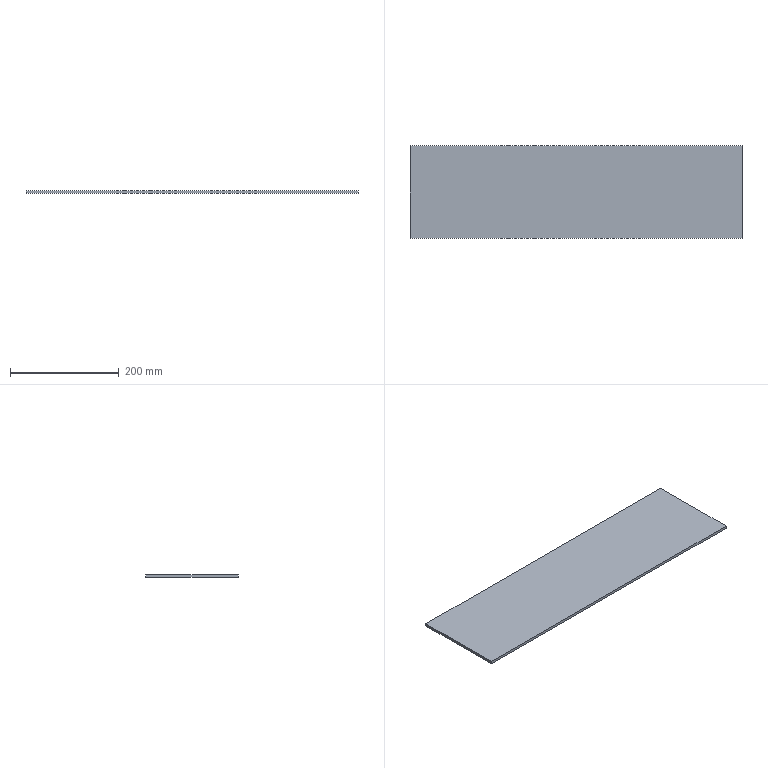Component | SolidWorks | CoverPlate5-1 | 1 solid | 6 faces | box 610 x 170 x 5 mm | volume 518500 mm3 | plane 6
build123d program:
from build123d import *

# Parameters (mm, degrees)
SKETCH1_W      = 610
SKETCH1_H      = 170
EXTRUDE1_DEPTH = 5


with BuildPart() as part:
    # Sketch1 → Extrude1 (new body)
    with BuildSketch(Plane.XY):
        Rectangle(SKETCH1_W, SKETCH1_H)
    extrude(amount=EXTRUDE1_DEPTH)


solid = part.part

# Placed as in the assembly
solid = solid.moved(Location((15, 530, -25), (0, 0, 0)))
STEP:
#1=COLOUR_RGB('',0.7922,0.8196,0.9333);
#2=FILL_AREA_STYLE_COLOUR('',#1);
#3=FILL_AREA_STYLE('',(#2));
#4=SURFACE_STYLE_FILL_AREA(#3);
#5=SURFACE_SIDE_STYLE('',(#4));
#6=SURFACE_STYLE_USAGE(.BOTH.,#5);
#7=PRESENTATION_STYLE_ASSIGNMENT((#6));
#8=CARTESIAN_POINT('',(12.598,17.52,-0.9843));
#9=VERTEX_POINT('',#8);
#10=CARTESIAN_POINT('',(12.598,24.213,-0.9843));
#11=VERTEX_POINT('',#10);
#12=CARTESIAN_POINT('',(12.598,24.213,-0.9843));
#13=DIRECTION('',(0.,1.,0.));
#14=VECTOR('',#13,39.37);
#15=LINE('',#12,#14);
#16=EDGE_CURVE('',#9,#11,#15,.T.);
#17=ORIENTED_EDGE('',*,*,#16,.T.);
#18=CARTESIAN_POINT('',(12.598,24.213,-0.7874));
#19=VERTEX_POINT('',#18);
#20=CARTESIAN_POINT('',(12.598,24.213,-0.7874));
#21=DIRECTION('',(0.,0.,-1.));
#22=VECTOR('',#21,39.37);
#23=LINE('',#20,#22);
#24=EDGE_CURVE('',#19,#11,#23,.T.);
#25=ORIENTED_EDGE('',*,*,#24,.F.);
#26=CARTESIAN_POINT('',(12.598,17.52,-0.7874));
#27=VERTEX_POINT('',#26);
#28=CARTESIAN_POINT('',(12.598,24.213,-0.7874));
#29=DIRECTION('',(0.,1.,0.));
#30=VECTOR('',#29,39.37);
#31=LINE('',#28,#30);
#32=EDGE_CURVE('',#27,#19,#31,.T.);
#33=ORIENTED_EDGE('',*,*,#32,.F.);
#34=CARTESIAN_POINT('',(12.598,17.52,-0.7874));
#35=DIRECTION('',(0.,0.,-1.));
#36=VECTOR('',#35,39.37);
#37=LINE('',#34,#36);
#38=EDGE_CURVE('',#27,#9,#37,.T.);
#39=ORIENTED_EDGE('',*,*,#38,.T.);
#40=EDGE_LOOP('',(#17,#25,#33,#39));
#41=FACE_OUTER_BOUND('',#40,.T.);
#42=CARTESIAN_POINT('',(12.598,24.213,-0.7874));
#43=DIRECTION('',(-1.,0.,0.));
#44=DIRECTION('',(0.,0.,1.));
#45=AXIS2_PLACEMENT_3D('',#42,#43,#44);
#46=PLANE('',#45);
#47=ADVANCED_FACE('',(#41),#46,.F.);
#48=CARTESIAN_POINT('',(-11.417,24.213,-0.9843));
#49=VERTEX_POINT('',#48);
#50=CARTESIAN_POINT('',(-11.417,24.213,-0.9843));
#51=DIRECTION('',(-1.,0.,0.));
#52=VECTOR('',#51,39.37);
#53=LINE('',#50,#52);
#54=EDGE_CURVE('',#11,#49,#53,.T.);
#55=ORIENTED_EDGE('',*,*,#54,.T.);
#56=CARTESIAN_POINT('',(-11.417,24.213,-0.7874));
#57=VERTEX_POINT('',#56);
#58=CARTESIAN_POINT('',(-11.417,24.213,-0.7874));
#59=DIRECTION('',(0.,0.,-1.));
#60=VECTOR('',#59,39.37);
#61=LINE('',#58,#60);
#62=EDGE_CURVE('',#57,#49,#61,.T.);
#63=ORIENTED_EDGE('',*,*,#62,.F.);
#64=CARTESIAN_POINT('',(-11.417,24.213,-0.7874));
#65=DIRECTION('',(-1.,0.,0.));
#66=VECTOR('',#65,39.37);
#67=LINE('',#64,#66);
#68=EDGE_CURVE('',#19,#57,#67,.T.);
#69=ORIENTED_EDGE('',*,*,#68,.F.);
#70=ORIENTED_EDGE('',*,*,#24,.T.);
#71=EDGE_LOOP('',(#55,#63,#69,#70));
#72=FACE_OUTER_BOUND('',#71,.T.);
#73=CARTESIAN_POINT('',(-11.417,24.213,-0.7874));
#74=DIRECTION('',(0.,-1.,0.));
#75=DIRECTION('',(0.,0.,-1.));
#76=AXIS2_PLACEMENT_3D('',#73,#74,#75);
#77=PLANE('',#76);
#78=ADVANCED_FACE('',(#72),#77,.F.);
#79=CARTESIAN_POINT('',(-11.417,17.52,-0.9843));
#80=VERTEX_POINT('',#79);
#81=CARTESIAN_POINT('',(-11.417,24.213,-0.9843));
#82=DIRECTION('',(-0.,-1.,0.));
#83=VECTOR('',#82,39.37);
#84=LINE('',#81,#83);
#85=EDGE_CURVE('',#49,#80,#84,.T.);
#86=ORIENTED_EDGE('',*,*,#85,.T.);
#87=CARTESIAN_POINT('',(-11.417,17.52,-0.7874));
#88=VERTEX_POINT('',#87);
#89=CARTESIAN_POINT('',(-11.417,17.52,-0.7874));
#90=DIRECTION('',(0.,0.,-1.));
#91=VECTOR('',#90,39.37);
#92=LINE('',#89,#91);
#93=EDGE_CURVE('',#88,#80,#92,.T.);
#94=ORIENTED_EDGE('',*,*,#93,.F.);
#95=CARTESIAN_POINT('',(-11.417,24.213,-0.7874));
#96=DIRECTION('',(-0.,-1.,0.));
#97=VECTOR('',#96,39.37);
#98=LINE('',#95,#97);
#99=EDGE_CURVE('',#57,#88,#98,.T.);
#100=ORIENTED_EDGE('',*,*,#99,.F.);
#101=ORIENTED_EDGE('',*,*,#62,.T.);
#102=EDGE_LOOP('',(#86,#94,#100,#101));
#103=FACE_OUTER_BOUND('',#102,.T.);
#104=CARTESIAN_POINT('',(-11.417,24.213,-0.7874));
#105=DIRECTION('',(1.,-0.,0.));
#106=DIRECTION('',(0.,1.,0.));
#107=AXIS2_PLACEMENT_3D('',#104,#105,#106);
#108=PLANE('',#107);
#109=ADVANCED_FACE('',(#103),#108,.F.);
#110=CARTESIAN_POINT('',(-11.417,17.52,-0.9843));
#111=DIRECTION('',(1.,0.,0.));
#112=VECTOR('',#111,39.37);
#113=LINE('',#110,#112);
#114=EDGE_CURVE('',#80,#9,#113,.T.);
#115=ORIENTED_EDGE('',*,*,#114,.T.);
#116=ORIENTED_EDGE('',*,*,#38,.F.);
#117=CARTESIAN_POINT('',(-11.417,17.52,-0.7874));
#118=DIRECTION('',(1.,0.,0.));
#119=VECTOR('',#118,39.37);
#120=LINE('',#117,#119);
#121=EDGE_CURVE('',#88,#27,#120,.T.);
#122=ORIENTED_EDGE('',*,*,#121,.F.);
#123=ORIENTED_EDGE('',*,*,#93,.T.);
#124=EDGE_LOOP('',(#115,#116,#122,#123));
#125=FACE_OUTER_BOUND('',#124,.T.);
#126=CARTESIAN_POINT('',(-11.417,17.52,-0.7874));
#127=DIRECTION('',(0.,1.,0.));
#128=DIRECTION('',(0.,0.,1.));
#129=AXIS2_PLACEMENT_3D('',#126,#127,#128);
#130=PLANE('',#129);
#131=ADVANCED_FACE('',(#125),#130,.F.);
#132=ORIENTED_EDGE('',*,*,#32,.T.);
#133=ORIENTED_EDGE('',*,*,#68,.T.);
#134=ORIENTED_EDGE('',*,*,#99,.T.);
#135=ORIENTED_EDGE('',*,*,#121,.T.);
#136=EDGE_LOOP('',(#132,#133,#134,#135));
#137=FACE_OUTER_BOUND('',#136,.T.);
#138=CARTESIAN_POINT('',(0.5906,20.866,-0.7874));
#139=DIRECTION('',(0.,0.,1.));
#140=DIRECTION('',(1.,0.,0.));
#141=AXIS2_PLACEMENT_3D('',#138,#139,#140);
#142=PLANE('',#141);
#143=ADVANCED_FACE('',(#137),#142,.T.);
#144=ORIENTED_EDGE('',*,*,#16,.F.);
#145=ORIENTED_EDGE('',*,*,#114,.F.);
#146=ORIENTED_EDGE('',*,*,#85,.F.);
#147=ORIENTED_EDGE('',*,*,#54,.F.);
#148=EDGE_LOOP('',(#144,#145,#146,#147));
#149=FACE_OUTER_BOUND('',#148,.T.);
#150=CARTESIAN_POINT('',(0.5906,20.866,-0.9843));
#151=DIRECTION('',(0.,0.,1.));
#152=DIRECTION('',(1.,0.,0.));
#153=AXIS2_PLACEMENT_3D('',#150,#151,#152);
#154=PLANE('',#153);
#155=ADVANCED_FACE('',(#149),#154,.F.);
#156=CLOSED_SHELL('',(#47,#78,#109,#131,#143,#155));
#157=MANIFOLD_SOLID_BREP('',#156);
#158=STYLED_ITEM('',(#7),#157);
#159=(LENGTH_UNIT()NAMED_UNIT(*)SI_UNIT($,.METRE.));
#160=LENGTH_MEASURE_WITH_UNIT(LENGTH_MEASURE(0.0254),#159);
#161=DIMENSIONAL_EXPONENTS(1.,0.,0.,0.,0.,0.,0.);
#162=(CONVERSION_BASED_UNIT('',#160)LENGTH_UNIT()NAMED_UNIT(#161));
#163=UNCERTAINTY_MEASURE_WITH_UNIT(LENGTH_MEASURE(0.00001),#162,'','');
#164=(NAMED_UNIT(*)PLANE_ANGLE_UNIT()SI_UNIT($,.RADIAN.));
#165=(NAMED_UNIT(*)SI_UNIT($,.STERADIAN.)SOLID_ANGLE_UNIT());
#166=(GEOMETRIC_REPRESENTATION_CONTEXT(3)GLOBAL_UNCERTAINTY_ASSIGNED_CONTEXT((#163))GLOBAL_UNIT_ASSIGNED_CONTEXT((#162,#164,#165))REPRESENTATION_CONTEXT('',''));
#167=MECHANICAL_DESIGN_GEOMETRIC_PRESENTATION_REPRESENTATION('',(#158),#166);
#168=PRESENTATION_LAYER_ASSIGNMENT('','',(#158));
#169=CARTESIAN_POINT('',(0.,0.,0.));
#170=DIRECTION('',(0.,0.,1.));
#171=DIRECTION('',(1.,0.,0.));
#172=AXIS2_PLACEMENT_3D('',#169,#170,#171);
#173=(LENGTH_UNIT()NAMED_UNIT(*)SI_UNIT($,.METRE.));
#174=LENGTH_MEASURE_WITH_UNIT(LENGTH_MEASURE(0.0254),#173);
#175=DIMENSIONAL_EXPONENTS(1.,0.,0.,0.,0.,0.,0.);
#176=(CONVERSION_BASED_UNIT('',#174)LENGTH_UNIT()NAMED_UNIT(#175));
#177=UNCERTAINTY_MEASURE_WITH_UNIT(LENGTH_MEASURE(0.00001),#176,'','');
#178=(NAMED_UNIT(*)PLANE_ANGLE_UNIT()SI_UNIT($,.RADIAN.));
#179=(NAMED_UNIT(*)SI_UNIT($,.STERADIAN.)SOLID_ANGLE_UNIT());
#180=(GEOMETRIC_REPRESENTATION_CONTEXT(3)GLOBAL_UNCERTAINTY_ASSIGNED_CONTEXT((#177))GLOBAL_UNIT_ASSIGNED_CONTEXT((#176,#178,#179))REPRESENTATION_CONTEXT('',''));
#181=ADVANCED_BREP_SHAPE_REPRESENTATION('',(#157,#172),#180);